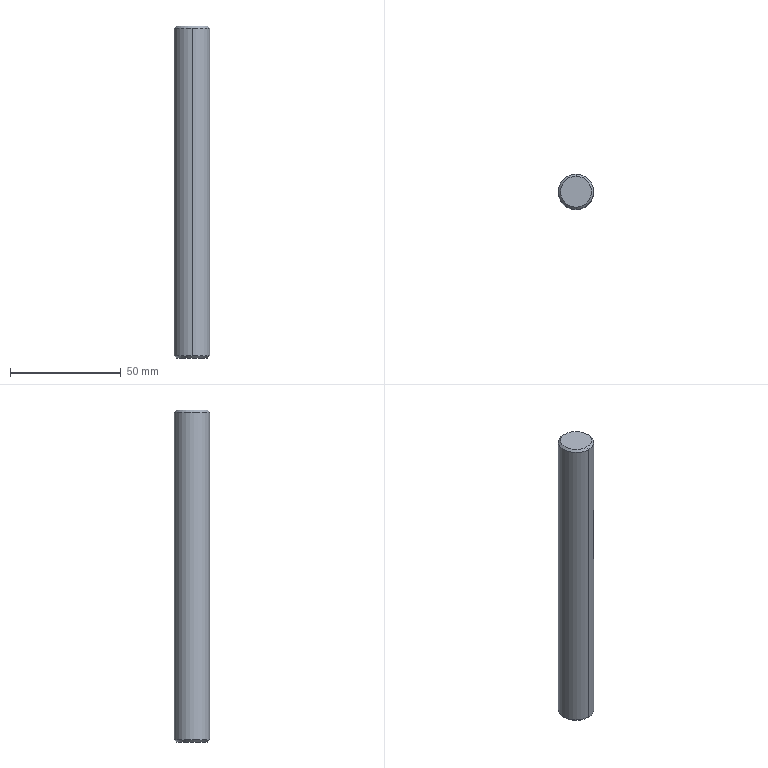Component | SolidWorks | CameraAssembly-1_GuideAxis16-1 | 1 solid | 8 faces | box 16 x 16 x 150 mm | volume 30111 mm3 | cone 4 | cylinder 2 | plane 2 | commonest cylinder face diameters 16 x2 | material Plain Carbon Steel
build123d program:
from build123d import *

# Parameters (mm, degrees)
SKETCH1_R           = 8
BOSS_EXTRUDE1_DEPTH = 150
CHAMFER1_SIZE       = 1


with BuildPart() as part:
    # Sketch1 → Boss-Extrude1 (new body)
    with BuildSketch(Plane.XY):
        Circle(SKETCH1_R)
    extrude(amount=BOSS_EXTRUDE1_DEPTH)

    # Chamfer1
    chamfer1_edges = [part.edges().sort_by_distance(p)[0] for p in [
        (-8, 0, 0),
        (-8, 0, 150),
    ]]
    chamfer(chamfer1_edges, length=CHAMFER1_SIZE)


solid = part.part

# Placed as in the assembly
solid = solid.moved(Location((-119.666, 150.264, -327.5), (0, 0, 0)))
STEP:
#1=CARTESIAN_POINT('',(-4.711,6.191,-12.894));
#2=VERTEX_POINT('',#1);
#3=CARTESIAN_POINT('',(-4.711,5.64,-12.894));
#4=VERTEX_POINT('',#3);
#5=CARTESIAN_POINT('',(-4.711,5.916,-12.894));
#6=DIRECTION('',(-0.,-0.,-1.));
#7=DIRECTION('',(0.,1.,0.));
#8=AXIS2_PLACEMENT_3D('',#5,#6,#7);
#9=CIRCLE('',#8,0.2756);
#10=EDGE_CURVE('',#2,#4,#9,.T.);
#11=ORIENTED_EDGE('',*,*,#10,.F.);
#12=CARTESIAN_POINT('',(-4.711,6.231,-12.854));
#13=VERTEX_POINT('',#12);
#14=CARTESIAN_POINT('',(-4.711,6.191,-12.894));
#15=DIRECTION('',(0.,0.7071,0.7071));
#16=VECTOR('',#15,39.37);
#17=LINE('',#14,#16);
#18=EDGE_CURVE('',#2,#13,#17,.T.);
#19=ORIENTED_EDGE('',*,*,#18,.T.);
#20=CARTESIAN_POINT('',(-4.711,5.601,-12.854));
#21=VERTEX_POINT('',#20);
#22=CARTESIAN_POINT('',(-4.711,5.916,-12.854));
#23=DIRECTION('',(0.,0.,1.));
#24=DIRECTION('',(0.,1.,0.));
#25=AXIS2_PLACEMENT_3D('',#22,#23,#24);
#26=CIRCLE('',#25,0.315);
#27=EDGE_CURVE('',#21,#13,#26,.T.);
#28=ORIENTED_EDGE('',*,*,#27,.F.);
#29=CARTESIAN_POINT('',(-4.711,5.64,-12.894));
#30=DIRECTION('',(-0.,-0.7071,0.7071));
#31=VECTOR('',#30,39.37);
#32=LINE('',#29,#31);
#33=EDGE_CURVE('',#4,#21,#32,.T.);
#34=ORIENTED_EDGE('',*,*,#33,.F.);
#35=EDGE_LOOP('',(#11,#19,#28,#34));
#36=FACE_OUTER_BOUND('',#35,.T.);
#37=CARTESIAN_POINT('',(-4.711,5.916,-12.894));
#38=DIRECTION('',(0.,0.,1.));
#39=DIRECTION('',(0.,-1.,0.));
#40=AXIS2_PLACEMENT_3D('',#37,#38,#39);
#41=CONICAL_SURFACE('',#40,0.2756,0.7854);
#42=ADVANCED_FACE('',(#36),#41,.T.);
#43=CARTESIAN_POINT('',(-4.711,5.64,-6.988));
#44=VERTEX_POINT('',#43);
#45=CARTESIAN_POINT('',(-4.711,6.191,-6.988));
#46=VERTEX_POINT('',#45);
#47=CARTESIAN_POINT('',(-4.711,5.916,-6.988));
#48=DIRECTION('',(0.,0.,1.));
#49=DIRECTION('',(0.,1.,0.));
#50=AXIS2_PLACEMENT_3D('',#47,#48,#49);
#51=CIRCLE('',#50,0.2756);
#52=EDGE_CURVE('',#44,#46,#51,.T.);
#53=ORIENTED_EDGE('',*,*,#52,.F.);
#54=CARTESIAN_POINT('',(-4.711,5.601,-7.028));
#55=VERTEX_POINT('',#54);
#56=CARTESIAN_POINT('',(-4.711,5.601,-7.028));
#57=DIRECTION('',(-0.,-0.7071,-0.7071));
#58=VECTOR('',#57,39.37);
#59=LINE('',#56,#58);
#60=EDGE_CURVE('',#44,#55,#59,.T.);
#61=ORIENTED_EDGE('',*,*,#60,.T.);
#62=CARTESIAN_POINT('',(-4.711,6.231,-7.028));
#63=VERTEX_POINT('',#62);
#64=CARTESIAN_POINT('',(-4.711,5.916,-7.028));
#65=DIRECTION('',(-0.,-0.,-1.));
#66=DIRECTION('',(0.,1.,0.));
#67=AXIS2_PLACEMENT_3D('',#64,#65,#66);
#68=CIRCLE('',#67,0.315);
#69=EDGE_CURVE('',#63,#55,#68,.T.);
#70=ORIENTED_EDGE('',*,*,#69,.F.);
#71=CARTESIAN_POINT('',(-4.711,6.231,-7.028));
#72=DIRECTION('',(0.,0.7071,-0.7071));
#73=VECTOR('',#72,39.37);
#74=LINE('',#71,#73);
#75=EDGE_CURVE('',#46,#63,#74,.T.);
#76=ORIENTED_EDGE('',*,*,#75,.F.);
#77=EDGE_LOOP('',(#53,#61,#70,#76));
#78=FACE_OUTER_BOUND('',#77,.T.);
#79=CARTESIAN_POINT('',(-4.711,5.916,-7.028));
#80=DIRECTION('',(-0.,-0.,-1.));
#81=DIRECTION('',(0.,1.,0.));
#82=AXIS2_PLACEMENT_3D('',#79,#80,#81);
#83=CONICAL_SURFACE('',#82,0.315,0.7854);
#84=ADVANCED_FACE('',(#78),#83,.T.);
#85=ORIENTED_EDGE('',*,*,#27,.T.);
#86=CARTESIAN_POINT('',(-4.711,6.231,-12.894));
#87=DIRECTION('',(0.,0.,1.));
#88=VECTOR('',#87,39.37);
#89=LINE('',#86,#88);
#90=EDGE_CURVE('',#13,#63,#89,.T.);
#91=ORIENTED_EDGE('',*,*,#90,.T.);
#92=ORIENTED_EDGE('',*,*,#69,.T.);
#93=CARTESIAN_POINT('',(-4.711,5.601,-12.894));
#94=DIRECTION('',(0.,0.,1.));
#95=VECTOR('',#94,39.37);
#96=LINE('',#93,#95);
#97=EDGE_CURVE('',#21,#55,#96,.T.);
#98=ORIENTED_EDGE('',*,*,#97,.F.);
#99=EDGE_LOOP('',(#85,#91,#92,#98));
#100=FACE_OUTER_BOUND('',#99,.T.);
#101=CARTESIAN_POINT('',(-4.711,5.916,-12.894));
#102=DIRECTION('',(0.,0.,1.));
#103=DIRECTION('',(0.,-1.,0.));
#104=AXIS2_PLACEMENT_3D('',#101,#102,#103);
#105=CYLINDRICAL_SURFACE('',#104,0.315);
#106=ADVANCED_FACE('',(#100),#105,.T.);
#107=ORIENTED_EDGE('',*,*,#90,.F.);
#108=CARTESIAN_POINT('',(-4.711,5.916,-12.854));
#109=DIRECTION('',(0.,0.,1.));
#110=DIRECTION('',(0.,1.,0.));
#111=AXIS2_PLACEMENT_3D('',#108,#109,#110);
#112=CIRCLE('',#111,0.315);
#113=EDGE_CURVE('',#13,#21,#112,.T.);
#114=ORIENTED_EDGE('',*,*,#113,.T.);
#115=ORIENTED_EDGE('',*,*,#97,.T.);
#116=CARTESIAN_POINT('',(-4.711,5.916,-7.028));
#117=DIRECTION('',(-0.,-0.,-1.));
#118=DIRECTION('',(0.,1.,0.));
#119=AXIS2_PLACEMENT_3D('',#116,#117,#118);
#120=CIRCLE('',#119,0.315);
#121=EDGE_CURVE('',#55,#63,#120,.T.);
#122=ORIENTED_EDGE('',*,*,#121,.T.);
#123=EDGE_LOOP('',(#107,#114,#115,#122));
#124=FACE_OUTER_BOUND('',#123,.T.);
#125=CARTESIAN_POINT('',(-4.711,5.916,-12.894));
#126=DIRECTION('',(0.,0.,1.));
#127=DIRECTION('',(0.,-1.,0.));
#128=AXIS2_PLACEMENT_3D('',#125,#126,#127);
#129=CYLINDRICAL_SURFACE('',#128,0.315);
#130=ADVANCED_FACE('',(#124),#129,.T.);
#131=CARTESIAN_POINT('',(-4.711,5.916,-12.894));
#132=DIRECTION('',(-0.,-0.,-1.));
#133=DIRECTION('',(0.,1.,0.));
#134=AXIS2_PLACEMENT_3D('',#131,#132,#133);
#135=CIRCLE('',#134,0.2756);
#136=EDGE_CURVE('',#4,#2,#135,.T.);
#137=ORIENTED_EDGE('',*,*,#136,.T.);
#138=ORIENTED_EDGE('',*,*,#10,.T.);
#139=EDGE_LOOP('',(#137,#138));
#140=FACE_OUTER_BOUND('',#139,.T.);
#141=CARTESIAN_POINT('',(-4.711,5.916,-12.894));
#142=DIRECTION('',(-0.,-0.,-1.));
#143=DIRECTION('',(0.,1.,-0.));
#144=AXIS2_PLACEMENT_3D('',#141,#142,#143);
#145=PLANE('',#144);
#146=ADVANCED_FACE('',(#140),#145,.T.);
#147=CARTESIAN_POINT('',(-4.711,5.916,-6.988));
#148=DIRECTION('',(0.,0.,1.));
#149=DIRECTION('',(0.,1.,0.));
#150=AXIS2_PLACEMENT_3D('',#147,#148,#149);
#151=CIRCLE('',#150,0.2756);
#152=EDGE_CURVE('',#46,#44,#151,.T.);
#153=ORIENTED_EDGE('',*,*,#152,.T.);
#154=ORIENTED_EDGE('',*,*,#52,.T.);
#155=EDGE_LOOP('',(#153,#154));
#156=FACE_OUTER_BOUND('',#155,.T.);
#157=CARTESIAN_POINT('',(-4.711,5.916,-6.988));
#158=DIRECTION('',(-0.,-0.,-1.));
#159=DIRECTION('',(0.,1.,-0.));
#160=AXIS2_PLACEMENT_3D('',#157,#158,#159);
#161=PLANE('',#160);
#162=ADVANCED_FACE('',(#156),#161,.F.);
#163=ORIENTED_EDGE('',*,*,#60,.F.);
#164=ORIENTED_EDGE('',*,*,#152,.F.);
#165=ORIENTED_EDGE('',*,*,#75,.T.);
#166=ORIENTED_EDGE('',*,*,#121,.F.);
#167=EDGE_LOOP('',(#163,#164,#165,#166));
#168=FACE_OUTER_BOUND('',#167,.T.);
#169=CARTESIAN_POINT('',(-4.711,5.916,-7.028));
#170=DIRECTION('',(-0.,-0.,-1.));
#171=DIRECTION('',(0.,1.,0.));
#172=AXIS2_PLACEMENT_3D('',#169,#170,#171);
#173=CONICAL_SURFACE('',#172,0.315,0.7854);
#174=ADVANCED_FACE('',(#168),#173,.T.);
#175=ORIENTED_EDGE('',*,*,#18,.F.);
#176=ORIENTED_EDGE('',*,*,#136,.F.);
#177=ORIENTED_EDGE('',*,*,#33,.T.);
#178=ORIENTED_EDGE('',*,*,#113,.F.);
#179=EDGE_LOOP('',(#175,#176,#177,#178));
#180=FACE_OUTER_BOUND('',#179,.T.);
#181=CARTESIAN_POINT('',(-4.711,5.916,-12.894));
#182=DIRECTION('',(0.,0.,1.));
#183=DIRECTION('',(0.,-1.,0.));
#184=AXIS2_PLACEMENT_3D('',#181,#182,#183);
#185=CONICAL_SURFACE('',#184,0.2756,0.7854);
#186=ADVANCED_FACE('',(#180),#185,.T.);
#187=CLOSED_SHELL('',(#42,#84,#106,#130,#146,#162,#174,#186));
#188=MANIFOLD_SOLID_BREP('',#187);
#189=CARTESIAN_POINT('',(0.,0.,0.));
#190=DIRECTION('',(0.,0.,1.));
#191=DIRECTION('',(1.,0.,0.));
#192=AXIS2_PLACEMENT_3D('',#189,#190,#191);
#193=(LENGTH_UNIT()NAMED_UNIT(*)SI_UNIT($,.METRE.));
#194=LENGTH_MEASURE_WITH_UNIT(LENGTH_MEASURE(0.0254),#193);
#195=DIMENSIONAL_EXPONENTS(1.,0.,0.,0.,0.,0.,0.);
#196=(CONVERSION_BASED_UNIT('',#194)LENGTH_UNIT()NAMED_UNIT(#195));
#197=UNCERTAINTY_MEASURE_WITH_UNIT(LENGTH_MEASURE(0.00001),#196,'','');
#198=(NAMED_UNIT(*)PLANE_ANGLE_UNIT()SI_UNIT($,.RADIAN.));
#199=(NAMED_UNIT(*)SI_UNIT($,.STERADIAN.)SOLID_ANGLE_UNIT());
#200=(GEOMETRIC_REPRESENTATION_CONTEXT(3)GLOBAL_UNCERTAINTY_ASSIGNED_CONTEXT((#197))GLOBAL_UNIT_ASSIGNED_CONTEXT((#196,#198,#199))REPRESENTATION_CONTEXT('',''));
#201=ADVANCED_BREP_SHAPE_REPRESENTATION('',(#188,#192),#200);
#202=COLOUR_RGB('',0.7922,0.8196,0.9333);
#203=FILL_AREA_STYLE_COLOUR('',#202);
#204=FILL_AREA_STYLE('',(#203));
#205=SURFACE_STYLE_FILL_AREA(#204);
#206=SURFACE_SIDE_STYLE('',(#205));
#207=SURFACE_STYLE_USAGE(.BOTH.,#206);
#208=PRESENTATION_STYLE_ASSIGNMENT((#207));
#209=STYLED_ITEM('',(#208),#188);
#210=PRESENTATION_LAYER_ASSIGNMENT('','',(#209));
#211=(LENGTH_UNIT()NAMED_UNIT(*)SI_UNIT($,.METRE.));
#212=LENGTH_MEASURE_WITH_UNIT(LENGTH_MEASURE(0.0254),#211);
#213=DIMENSIONAL_EXPONENTS(1.,0.,0.,0.,0.,0.,0.);
#214=(CONVERSION_BASED_UNIT('',#212)LENGTH_UNIT()NAMED_UNIT(#213));
#215=UNCERTAINTY_MEASURE_WITH_UNIT(LENGTH_MEASURE(0.00001),#214,'','');
#216=(NAMED_UNIT(*)PLANE_ANGLE_UNIT()SI_UNIT($,.RADIAN.));
#217=(NAMED_UNIT(*)SI_UNIT($,.STERADIAN.)SOLID_ANGLE_UNIT());
#218=(GEOMETRIC_REPRESENTATION_CONTEXT(3)GLOBAL_UNCERTAINTY_ASSIGNED_CONTEXT((#215))GLOBAL_UNIT_ASSIGNED_CONTEXT((#214,#216,#217))REPRESENTATION_CONTEXT('',''));
#219=MECHANICAL_DESIGN_GEOMETRIC_PRESENTATION_REPRESENTATION('',(#209),#218);